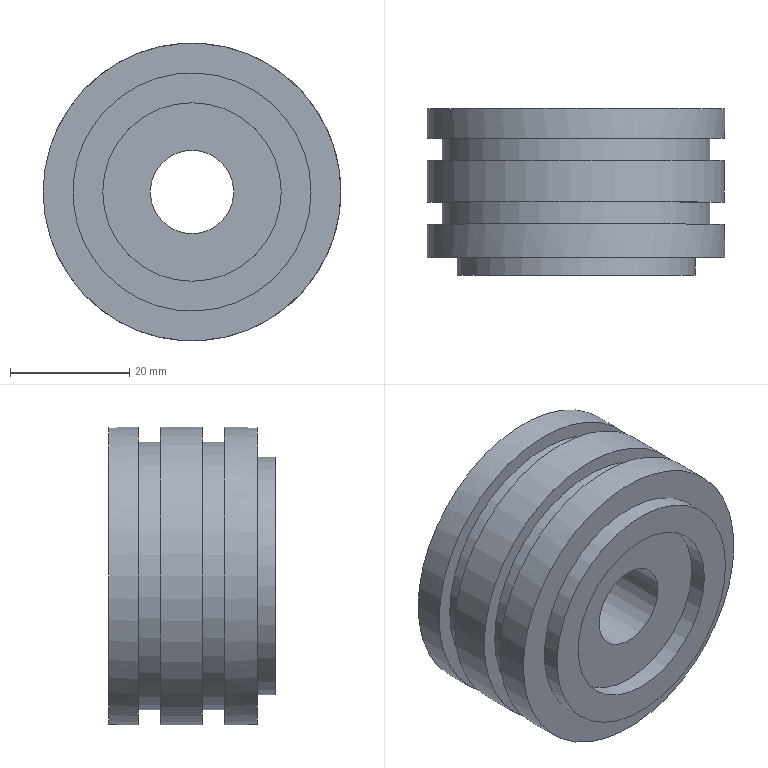Component | NX | PISTON | 1 solid | 18 faces | box 50 x 28 x 50 mm | volume 29970 mm3 | plane 9 | cylinder 8 | cone 1 | commonest cylinder face diameters 50 x3 45 x2 14 x1 40 x1 30 x1
STEP:
#1=CARTESIAN_POINT('',(0.,0.,0.));
#2=DIRECTION('',(0.,0.,1.));
#3=DIRECTION('',(1.,0.,0.));
#4=AXIS2_PLACEMENT_3D('',#1,#2,#3);
#5=CARTESIAN_POINT('',(-25.,44.,43.));
#6=VERTEX_POINT('',#5);
#7=CARTESIAN_POINT('',(25.,44.,43.));
#8=VERTEX_POINT('',#7);
#9=CARTESIAN_POINT('',(-0.,44.,43.));
#10=DIRECTION('',(0.,-1.,0.));
#11=DIRECTION('',(1.,0.,0.));
#12=AXIS2_PLACEMENT_3D('',#9,#10,#11);
#13=CIRCLE('',#12,25.);
#14=CARTESIAN_POINT('',(-0.,44.,43.));
#15=DIRECTION('',(0.,1.,0.));
#16=DIRECTION('',(-1.,0.,0.));
#17=AXIS2_PLACEMENT_3D('',#14,#15,#16);
#18=CYLINDRICAL_SURFACE('',#17,25.);
#19=CARTESIAN_POINT('',(9.425,0.));
#20=DIRECTION('',(-1.,0.));
#21=VECTOR('',#20,1.);
#22=LINE('',#19,#21);
#23=(GEOMETRIC_REPRESENTATION_CONTEXT(2)PARAMETRIC_REPRESENTATION_CONTEXT()REPRESENTATION_CONTEXT('',''));
#24=DEFINITIONAL_REPRESENTATION('',(#22),#23);
#25=PCURVE('',#18,#24);
#26=CARTESIAN_POINT('',(-0.,44.,43.));
#27=DIRECTION('',(0.,-1.,0.));
#28=DIRECTION('',(1.,0.,0.));
#29=AXIS2_PLACEMENT_3D('',#26,#27,#28);
#30=PLANE('',#29);
#31=CARTESIAN_POINT('',(0.,0.));
#32=DIRECTION('',(1.,0.));
#33=AXIS2_PLACEMENT_2D('',#31,#32);
#34=CIRCLE('',#33,25.);
#35=(GEOMETRIC_REPRESENTATION_CONTEXT(2)PARAMETRIC_REPRESENTATION_CONTEXT()REPRESENTATION_CONTEXT('',''));
#36=DEFINITIONAL_REPRESENTATION('',(#34),#35);
#37=PCURVE('',#30,#36);
#38=SURFACE_CURVE('',#13,(#25,#37),.PCURVE_S1.);
#39=EDGE_CURVE('',#6,#8,#38,.T.);
#40=ORIENTED_EDGE('',*,*,#39,.F.);
#41=CARTESIAN_POINT('',(-25.,49.6,43.));
#42=VERTEX_POINT('',#41);
#43=CARTESIAN_POINT('',(-25.,44.,43.));
#44=CARTESIAN_POINT('',(-25.,49.6,43.));
#45=B_SPLINE_CURVE_WITH_KNOTS('',1,(#43,#44),.UNSPECIFIED.,.F.,.F.,(2,2),(0.,5.6),.PIECEWISE_BEZIER_KNOTS.);
#46=CARTESIAN_POINT('',(6.283,0.));
#47=DIRECTION('',(0.,1.));
#48=VECTOR('',#47,1.);
#49=LINE('',#46,#48);
#50=(GEOMETRIC_REPRESENTATION_CONTEXT(2)PARAMETRIC_REPRESENTATION_CONTEXT()REPRESENTATION_CONTEXT('',''));
#51=DEFINITIONAL_REPRESENTATION('',(#49),#50);
#52=PCURVE('',#18,#51);
#53=CARTESIAN_POINT('',(0.,0.));
#54=DIRECTION('',(0.,1.));
#55=VECTOR('',#54,1.);
#56=LINE('',#53,#55);
#57=(GEOMETRIC_REPRESENTATION_CONTEXT(2)PARAMETRIC_REPRESENTATION_CONTEXT()REPRESENTATION_CONTEXT('',''));
#58=DEFINITIONAL_REPRESENTATION('',(#56),#57);
#59=PCURVE('',#18,#58);
#60=SEAM_CURVE('',#45,(#52,#59),.PCURVE_S1.);
#61=EDGE_CURVE('',#6,#42,#60,.T.);
#62=ORIENTED_EDGE('',*,*,#61,.T.);
#63=CARTESIAN_POINT('',(-0.,49.6,43.));
#64=DIRECTION('',(0.,1.,0.));
#65=DIRECTION('',(-1.,0.,0.));
#66=AXIS2_PLACEMENT_3D('',#63,#64,#65);
#67=CIRCLE('',#66,25.);
#68=CARTESIAN_POINT('',(0.,5.6));
#69=DIRECTION('',(1.,0.));
#70=VECTOR('',#69,1.);
#71=LINE('',#68,#70);
#72=(GEOMETRIC_REPRESENTATION_CONTEXT(2)PARAMETRIC_REPRESENTATION_CONTEXT()REPRESENTATION_CONTEXT('',''));
#73=DEFINITIONAL_REPRESENTATION('',(#71),#72);
#74=PCURVE('',#18,#73);
#75=CARTESIAN_POINT('',(-0.,49.6,43.));
#76=DIRECTION('',(0.,1.,0.));
#77=DIRECTION('',(-1.,0.,0.));
#78=AXIS2_PLACEMENT_3D('',#75,#76,#77);
#79=PLANE('',#78);
#80=CARTESIAN_POINT('',(0.,0.));
#81=DIRECTION('',(1.,0.));
#82=AXIS2_PLACEMENT_2D('',#80,#81);
#83=CIRCLE('',#82,25.);
#84=(GEOMETRIC_REPRESENTATION_CONTEXT(2)PARAMETRIC_REPRESENTATION_CONTEXT()REPRESENTATION_CONTEXT('',''));
#85=DEFINITIONAL_REPRESENTATION('',(#83),#84);
#86=PCURVE('',#79,#85);
#87=SURFACE_CURVE('',#67,(#74,#86),.PCURVE_S1.);
#88=EDGE_CURVE('',#42,#42,#87,.T.);
#89=ORIENTED_EDGE('',*,*,#88,.F.);
#90=ORIENTED_EDGE('',*,*,#61,.F.);
#91=CARTESIAN_POINT('',(-0.,44.,43.));
#92=DIRECTION('',(0.,-1.,0.));
#93=DIRECTION('',(1.,0.,0.));
#94=AXIS2_PLACEMENT_3D('',#91,#92,#93);
#95=CIRCLE('',#94,25.);
#96=CARTESIAN_POINT('',(3.142,0.));
#97=DIRECTION('',(-1.,0.));
#98=VECTOR('',#97,1.);
#99=LINE('',#96,#98);
#100=(GEOMETRIC_REPRESENTATION_CONTEXT(2)PARAMETRIC_REPRESENTATION_CONTEXT()REPRESENTATION_CONTEXT('',''));
#101=DEFINITIONAL_REPRESENTATION('',(#99),#100);
#102=PCURVE('',#18,#101);
#103=CARTESIAN_POINT('',(0.,0.));
#104=DIRECTION('',(1.,0.));
#105=AXIS2_PLACEMENT_2D('',#103,#104);
#106=CIRCLE('',#105,25.);
#107=(GEOMETRIC_REPRESENTATION_CONTEXT(2)PARAMETRIC_REPRESENTATION_CONTEXT()REPRESENTATION_CONTEXT('',''));
#108=DEFINITIONAL_REPRESENTATION('',(#106),#107);
#109=PCURVE('',#30,#108);
#110=SURFACE_CURVE('',#95,(#102,#109),.PCURVE_S1.);
#111=EDGE_CURVE('',#8,#6,#110,.T.);
#112=ORIENTED_EDGE('',*,*,#111,.F.);
#113=EDGE_LOOP('',(#40,#62,#89,#90,#112));
#114=FACE_BOUND('',#113,.T.);
#115=ADVANCED_FACE('',(#114),#18,.T.);
#116=CARTESIAN_POINT('',(-25.,53.3,43.));
#117=VERTEX_POINT('',#116);
#118=CARTESIAN_POINT('',(-0.,53.3,43.));
#119=DIRECTION('',(0.,1.,0.));
#120=DIRECTION('',(-1.,0.,0.));
#121=AXIS2_PLACEMENT_3D('',#118,#119,#120);
#122=CIRCLE('',#121,25.);
#123=CARTESIAN_POINT('',(-0.,44.,43.));
#124=DIRECTION('',(0.,1.,0.));
#125=DIRECTION('',(-1.,0.,0.));
#126=AXIS2_PLACEMENT_3D('',#123,#124,#125);
#127=CYLINDRICAL_SURFACE('',#126,25.);
#128=CARTESIAN_POINT('',(0.,9.3));
#129=DIRECTION('',(1.,0.));
#130=VECTOR('',#129,1.);
#131=LINE('',#128,#130);
#132=(GEOMETRIC_REPRESENTATION_CONTEXT(2)PARAMETRIC_REPRESENTATION_CONTEXT()REPRESENTATION_CONTEXT('',''));
#133=DEFINITIONAL_REPRESENTATION('',(#131),#132);
#134=PCURVE('',#127,#133);
#135=CARTESIAN_POINT('',(-0.,53.3,43.));
#136=DIRECTION('',(0.,1.,0.));
#137=DIRECTION('',(-1.,0.,0.));
#138=AXIS2_PLACEMENT_3D('',#135,#136,#137);
#139=PLANE('',#138);
#140=CARTESIAN_POINT('',(0.,0.));
#141=DIRECTION('',(1.,0.));
#142=AXIS2_PLACEMENT_2D('',#140,#141);
#143=CIRCLE('',#142,25.);
#144=(GEOMETRIC_REPRESENTATION_CONTEXT(2)PARAMETRIC_REPRESENTATION_CONTEXT()REPRESENTATION_CONTEXT('',''));
#145=DEFINITIONAL_REPRESENTATION('',(#143),#144);
#146=PCURVE('',#139,#145);
#147=SURFACE_CURVE('',#122,(#134,#146),.PCURVE_S1.);
#148=EDGE_CURVE('',#117,#117,#147,.T.);
#149=ORIENTED_EDGE('',*,*,#148,.T.);
#150=CARTESIAN_POINT('',(-25.,60.3,43.));
#151=VERTEX_POINT('',#150);
#152=CARTESIAN_POINT('',(-25.,53.3,43.));
#153=CARTESIAN_POINT('',(-25.,60.3,43.));
#154=B_SPLINE_CURVE_WITH_KNOTS('',1,(#152,#153),.UNSPECIFIED.,.F.,.F.,(2,2),(9.3,16.3),.PIECEWISE_BEZIER_KNOTS.);
#155=CARTESIAN_POINT('',(6.283,0.));
#156=DIRECTION('',(0.,1.));
#157=VECTOR('',#156,1.);
#158=LINE('',#155,#157);
#159=(GEOMETRIC_REPRESENTATION_CONTEXT(2)PARAMETRIC_REPRESENTATION_CONTEXT()REPRESENTATION_CONTEXT('',''));
#160=DEFINITIONAL_REPRESENTATION('',(#158),#159);
#161=PCURVE('',#127,#160);
#162=CARTESIAN_POINT('',(0.,0.));
#163=DIRECTION('',(0.,1.));
#164=VECTOR('',#163,1.);
#165=LINE('',#162,#164);
#166=(GEOMETRIC_REPRESENTATION_CONTEXT(2)PARAMETRIC_REPRESENTATION_CONTEXT()REPRESENTATION_CONTEXT('',''));
#167=DEFINITIONAL_REPRESENTATION('',(#165),#166);
#168=PCURVE('',#127,#167);
#169=SEAM_CURVE('',#154,(#161,#168),.PCURVE_S1.);
#170=EDGE_CURVE('',#117,#151,#169,.T.);
#171=ORIENTED_EDGE('',*,*,#170,.T.);
#172=CARTESIAN_POINT('',(-0.,60.3,43.));
#173=DIRECTION('',(0.,1.,0.));
#174=DIRECTION('',(-1.,0.,0.));
#175=AXIS2_PLACEMENT_3D('',#172,#173,#174);
#176=CIRCLE('',#175,25.);
#177=CARTESIAN_POINT('',(0.,16.3));
#178=DIRECTION('',(1.,0.));
#179=VECTOR('',#178,1.);
#180=LINE('',#177,#179);
#181=(GEOMETRIC_REPRESENTATION_CONTEXT(2)PARAMETRIC_REPRESENTATION_CONTEXT()REPRESENTATION_CONTEXT('',''));
#182=DEFINITIONAL_REPRESENTATION('',(#180),#181);
#183=PCURVE('',#127,#182);
#184=CARTESIAN_POINT('',(-0.,60.3,43.));
#185=DIRECTION('',(0.,1.,0.));
#186=DIRECTION('',(-1.,0.,0.));
#187=AXIS2_PLACEMENT_3D('',#184,#185,#186);
#188=PLANE('',#187);
#189=CARTESIAN_POINT('',(0.,0.));
#190=DIRECTION('',(1.,0.));
#191=AXIS2_PLACEMENT_2D('',#189,#190);
#192=CIRCLE('',#191,25.);
#193=(GEOMETRIC_REPRESENTATION_CONTEXT(2)PARAMETRIC_REPRESENTATION_CONTEXT()REPRESENTATION_CONTEXT('',''));
#194=DEFINITIONAL_REPRESENTATION('',(#192),#193);
#195=PCURVE('',#188,#194);
#196=SURFACE_CURVE('',#176,(#183,#195),.PCURVE_S1.);
#197=EDGE_CURVE('',#151,#151,#196,.T.);
#198=ORIENTED_EDGE('',*,*,#197,.F.);
#199=ORIENTED_EDGE('',*,*,#170,.F.);
#200=EDGE_LOOP('',(#149,#171,#198,#199));
#201=FACE_BOUND('',#200,.T.);
#202=ADVANCED_FACE('',(#201),#127,.T.);
#203=CARTESIAN_POINT('',(7.,44.,43.));
#204=VERTEX_POINT('',#203);
#205=CARTESIAN_POINT('',(-7.,44.,43.));
#206=VERTEX_POINT('',#205);
#207=CARTESIAN_POINT('',(-0.,44.,43.));
#208=DIRECTION('',(0.,1.,0.));
#209=DIRECTION('',(1.,0.,0.));
#210=AXIS2_PLACEMENT_3D('',#207,#208,#209);
#211=CIRCLE('',#210,7.);
#212=CARTESIAN_POINT('',(-0.,41.,43.));
#213=DIRECTION('',(0.,1.,0.));
#214=DIRECTION('',(-1.,0.,0.));
#215=AXIS2_PLACEMENT_3D('',#212,#213,#214);
#216=CYLINDRICAL_SURFACE('',#215,7.);
#217=CARTESIAN_POINT('',(3.142,3.));
#218=DIRECTION('',(1.,0.));
#219=VECTOR('',#218,1.);
#220=LINE('',#217,#219);
#221=(GEOMETRIC_REPRESENTATION_CONTEXT(2)PARAMETRIC_REPRESENTATION_CONTEXT()REPRESENTATION_CONTEXT('',''));
#222=DEFINITIONAL_REPRESENTATION('',(#220),#221);
#223=PCURVE('',#216,#222);
#224=CARTESIAN_POINT('',(-0.,44.,43.));
#225=DIRECTION('',(0.,-1.,0.));
#226=DIRECTION('',(1.,0.,0.));
#227=AXIS2_PLACEMENT_3D('',#224,#225,#226);
#228=PLANE('',#227);
#229=CARTESIAN_POINT('',(7.,0.));
#230=CARTESIAN_POINT('',(7.,-12.124));
#231=CARTESIAN_POINT('',(-3.5,-6.062));
#232=CARTESIAN_POINT('',(-14.,-0.));
#233=CARTESIAN_POINT('',(-3.5,6.062));
#234=CARTESIAN_POINT('',(7.,12.124));
#235=CARTESIAN_POINT('',(7.,0.));
#236=(BOUNDED_CURVE()B_SPLINE_CURVE(2,(#229,#230,#231,#232,#233,#234,#235),.UNSPECIFIED.,.T.,.F.)B_SPLINE_CURVE_WITH_KNOTS((1,2,2,2,2,1),(-2.094,0.,2.094,4.189,6.283,8.378),.UNSPECIFIED.)CURVE()GEOMETRIC_REPRESENTATION_ITEM()RATIONAL_B_SPLINE_CURVE((1.,0.5,1.,0.5,1.,0.5,1.))REPRESENTATION_ITEM(''));
#237=(GEOMETRIC_REPRESENTATION_CONTEXT(2)PARAMETRIC_REPRESENTATION_CONTEXT()REPRESENTATION_CONTEXT('',''));
#238=DEFINITIONAL_REPRESENTATION('',(#236),#237);
#239=PCURVE('',#228,#238);
#240=SURFACE_CURVE('',#211,(#223,#239),.PCURVE_S1.);
#241=EDGE_CURVE('',#204,#206,#240,.T.);
#242=ORIENTED_EDGE('',*,*,#241,.T.);
#243=CARTESIAN_POINT('',(-7.,54.,43.));
#244=VERTEX_POINT('',#243);
#245=CARTESIAN_POINT('',(-7.,44.,43.));
#246=CARTESIAN_POINT('',(-7.,54.,43.));
#247=B_SPLINE_CURVE_WITH_KNOTS('',1,(#245,#246),.UNSPECIFIED.,.F.,.F.,(2,2),(3.,13.),.PIECEWISE_BEZIER_KNOTS.);
#248=CARTESIAN_POINT('',(6.283,0.));
#249=DIRECTION('',(0.,1.));
#250=VECTOR('',#249,1.);
#251=LINE('',#248,#250);
#252=(GEOMETRIC_REPRESENTATION_CONTEXT(2)PARAMETRIC_REPRESENTATION_CONTEXT()REPRESENTATION_CONTEXT('',''));
#253=DEFINITIONAL_REPRESENTATION('',(#251),#252);
#254=PCURVE('',#216,#253);
#255=CARTESIAN_POINT('',(0.,0.));
#256=DIRECTION('',(0.,1.));
#257=VECTOR('',#256,1.);
#258=LINE('',#255,#257);
#259=(GEOMETRIC_REPRESENTATION_CONTEXT(2)PARAMETRIC_REPRESENTATION_CONTEXT()REPRESENTATION_CONTEXT('',''));
#260=DEFINITIONAL_REPRESENTATION('',(#258),#259);
#261=PCURVE('',#216,#260);
#262=SEAM_CURVE('',#247,(#254,#261),.PCURVE_S1.);
#263=EDGE_CURVE('',#206,#244,#262,.T.);
#264=ORIENTED_EDGE('',*,*,#263,.T.);
#265=CARTESIAN_POINT('',(-0.,54.,43.));
#266=DIRECTION('',(0.,-1.,0.));
#267=DIRECTION('',(-1.,0.,0.));
#268=AXIS2_PLACEMENT_3D('',#265,#266,#267);
#269=CIRCLE('',#268,7.);
#270=CARTESIAN_POINT('',(6.283,13.));
#271=DIRECTION('',(-1.,0.));
#272=VECTOR('',#271,1.);
#273=LINE('',#270,#272);
#274=(GEOMETRIC_REPRESENTATION_CONTEXT(2)PARAMETRIC_REPRESENTATION_CONTEXT()REPRESENTATION_CONTEXT('',''));
#275=DEFINITIONAL_REPRESENTATION('',(#273),#274);
#276=PCURVE('',#216,#275);
#277=CARTESIAN_POINT('',(-0.,54.,43.));
#278=DIRECTION('',(0.,1.,0.));
#279=DIRECTION('',(-1.,0.,0.));
#280=AXIS2_PLACEMENT_3D('',#277,#278,#279);
#281=PLANE('',#280);
#282=CARTESIAN_POINT('',(7.,0.));
#283=CARTESIAN_POINT('',(7.,-12.124));
#284=CARTESIAN_POINT('',(-3.5,-6.062));
#285=CARTESIAN_POINT('',(-14.,-0.));
#286=CARTESIAN_POINT('',(-3.5,6.062));
#287=CARTESIAN_POINT('',(7.,12.124));
#288=CARTESIAN_POINT('',(7.,0.));
#289=(BOUNDED_CURVE()B_SPLINE_CURVE(2,(#282,#283,#284,#285,#286,#287,#288),.UNSPECIFIED.,.T.,.F.)B_SPLINE_CURVE_WITH_KNOTS((1,2,2,2,2,1),(-2.094,0.,2.094,4.189,6.283,8.378),.UNSPECIFIED.)CURVE()GEOMETRIC_REPRESENTATION_ITEM()RATIONAL_B_SPLINE_CURVE((1.,0.5,1.,0.5,1.,0.5,1.))REPRESENTATION_ITEM(''));
#290=(GEOMETRIC_REPRESENTATION_CONTEXT(2)PARAMETRIC_REPRESENTATION_CONTEXT()REPRESENTATION_CONTEXT('',''));
#291=DEFINITIONAL_REPRESENTATION('',(#289),#290);
#292=PCURVE('',#281,#291);
#293=SURFACE_CURVE('',#269,(#276,#292),.PCURVE_S1.);
#294=EDGE_CURVE('',#244,#244,#293,.T.);
#295=ORIENTED_EDGE('',*,*,#294,.T.);
#296=ORIENTED_EDGE('',*,*,#263,.F.);
#297=CARTESIAN_POINT('',(-0.,44.,43.));
#298=DIRECTION('',(0.,1.,0.));
#299=DIRECTION('',(1.,0.,0.));
#300=AXIS2_PLACEMENT_3D('',#297,#298,#299);
#301=CIRCLE('',#300,7.);
#302=CARTESIAN_POINT('',(-3.142,3.));
#303=DIRECTION('',(1.,0.));
#304=VECTOR('',#303,1.);
#305=LINE('',#302,#304);
#306=(GEOMETRIC_REPRESENTATION_CONTEXT(2)PARAMETRIC_REPRESENTATION_CONTEXT()REPRESENTATION_CONTEXT('',''));
#307=DEFINITIONAL_REPRESENTATION('',(#305),#306);
#308=PCURVE('',#216,#307);
#309=CARTESIAN_POINT('',(7.,0.));
#310=CARTESIAN_POINT('',(7.,-12.124));
#311=CARTESIAN_POINT('',(-3.5,-6.062));
#312=CARTESIAN_POINT('',(-14.,-0.));
#313=CARTESIAN_POINT('',(-3.5,6.062));
#314=CARTESIAN_POINT('',(7.,12.124));
#315=CARTESIAN_POINT('',(7.,0.));
#316=(BOUNDED_CURVE()B_SPLINE_CURVE(2,(#309,#310,#311,#312,#313,#314,#315),.UNSPECIFIED.,.T.,.F.)B_SPLINE_CURVE_WITH_KNOTS((1,2,2,2,2,1),(-2.094,0.,2.094,4.189,6.283,8.378),.UNSPECIFIED.)CURVE()GEOMETRIC_REPRESENTATION_ITEM()RATIONAL_B_SPLINE_CURVE((1.,0.5,1.,0.5,1.,0.5,1.))REPRESENTATION_ITEM(''));
#317=(GEOMETRIC_REPRESENTATION_CONTEXT(2)PARAMETRIC_REPRESENTATION_CONTEXT()REPRESENTATION_CONTEXT('',''));
#318=DEFINITIONAL_REPRESENTATION('',(#316),#317);
#319=PCURVE('',#228,#318);
#320=SURFACE_CURVE('',#301,(#308,#319),.PCURVE_S1.);
#321=EDGE_CURVE('',#206,#204,#320,.T.);
#322=ORIENTED_EDGE('',*,*,#321,.T.);
#323=EDGE_LOOP('',(#242,#264,#295,#296,#322));
#324=FACE_BOUND('',#323,.F.);
#325=ADVANCED_FACE('',(#324),#216,.F.);
#326=CARTESIAN_POINT('',(-25.,64.,43.));
#327=VERTEX_POINT('',#326);
#328=CARTESIAN_POINT('',(-0.,64.,43.));
#329=DIRECTION('',(0.,1.,0.));
#330=DIRECTION('',(-1.,0.,0.));
#331=AXIS2_PLACEMENT_3D('',#328,#329,#330);
#332=CIRCLE('',#331,25.);
#333=CARTESIAN_POINT('',(-0.,44.,43.));
#334=DIRECTION('',(0.,1.,0.));
#335=DIRECTION('',(-1.,0.,0.));
#336=AXIS2_PLACEMENT_3D('',#333,#334,#335);
#337=CYLINDRICAL_SURFACE('',#336,25.);
#338=CARTESIAN_POINT('',(0.,20.));
#339=DIRECTION('',(1.,0.));
#340=VECTOR('',#339,1.);
#341=LINE('',#338,#340);
#342=(GEOMETRIC_REPRESENTATION_CONTEXT(2)PARAMETRIC_REPRESENTATION_CONTEXT()REPRESENTATION_CONTEXT('',''));
#343=DEFINITIONAL_REPRESENTATION('',(#341),#342);
#344=PCURVE('',#337,#343);
#345=CARTESIAN_POINT('',(-0.,64.,43.));
#346=DIRECTION('',(0.,1.,0.));
#347=DIRECTION('',(-1.,0.,0.));
#348=AXIS2_PLACEMENT_3D('',#345,#346,#347);
#349=PLANE('',#348);
#350=CARTESIAN_POINT('',(0.,0.));
#351=DIRECTION('',(1.,0.));
#352=AXIS2_PLACEMENT_2D('',#350,#351);
#353=CIRCLE('',#352,25.);
#354=(GEOMETRIC_REPRESENTATION_CONTEXT(2)PARAMETRIC_REPRESENTATION_CONTEXT()REPRESENTATION_CONTEXT('',''));
#355=DEFINITIONAL_REPRESENTATION('',(#353),#354);
#356=PCURVE('',#349,#355);
#357=SURFACE_CURVE('',#332,(#344,#356),.PCURVE_S1.);
#358=EDGE_CURVE('',#327,#327,#357,.T.);
#359=ORIENTED_EDGE('',*,*,#358,.T.);
#360=CARTESIAN_POINT('',(-25.,69.,43.));
#361=VERTEX_POINT('',#360);
#362=CARTESIAN_POINT('',(-25.,64.,43.));
#363=CARTESIAN_POINT('',(-25.,69.,43.));
#364=B_SPLINE_CURVE_WITH_KNOTS('',1,(#362,#363),.UNSPECIFIED.,.F.,.F.,(2,2),(20.,25.),.PIECEWISE_BEZIER_KNOTS.);
#365=CARTESIAN_POINT('',(6.283,0.));
#366=DIRECTION('',(0.,1.));
#367=VECTOR('',#366,1.);
#368=LINE('',#365,#367);
#369=(GEOMETRIC_REPRESENTATION_CONTEXT(2)PARAMETRIC_REPRESENTATION_CONTEXT()REPRESENTATION_CONTEXT('',''));
#370=DEFINITIONAL_REPRESENTATION('',(#368),#369);
#371=PCURVE('',#337,#370);
#372=CARTESIAN_POINT('',(0.,0.));
#373=DIRECTION('',(0.,1.));
#374=VECTOR('',#373,1.);
#375=LINE('',#372,#374);
#376=(GEOMETRIC_REPRESENTATION_CONTEXT(2)PARAMETRIC_REPRESENTATION_CONTEXT()REPRESENTATION_CONTEXT('',''));
#377=DEFINITIONAL_REPRESENTATION('',(#375),#376);
#378=PCURVE('',#337,#377);
#379=SEAM_CURVE('',#364,(#371,#378),.PCURVE_S1.);
#380=EDGE_CURVE('',#327,#361,#379,.T.);
#381=ORIENTED_EDGE('',*,*,#380,.T.);
#382=CARTESIAN_POINT('',(25.,69.,43.));
#383=VERTEX_POINT('',#382);
#384=CARTESIAN_POINT('',(-0.,69.,43.));
#385=DIRECTION('',(0.,-1.,0.));
#386=DIRECTION('',(1.,0.,0.));
#387=AXIS2_PLACEMENT_3D('',#384,#385,#386);
#388=CIRCLE('',#387,25.);
#389=CARTESIAN_POINT('',(9.425,25.));
#390=DIRECTION('',(-1.,0.));
#391=VECTOR('',#390,1.);
#392=LINE('',#389,#391);
#393=(GEOMETRIC_REPRESENTATION_CONTEXT(2)PARAMETRIC_REPRESENTATION_CONTEXT()REPRESENTATION_CONTEXT('',''));
#394=DEFINITIONAL_REPRESENTATION('',(#392),#393);
#395=PCURVE('',#337,#394);
#396=CARTESIAN_POINT('',(-0.,69.,43.));
#397=DIRECTION('',(0.,-1.,0.));
#398=DIRECTION('',(1.,0.,0.));
#399=AXIS2_PLACEMENT_3D('',#396,#397,#398);
#400=PLANE('',#399);
#401=CARTESIAN_POINT('',(0.,0.));
#402=DIRECTION('',(1.,0.));
#403=AXIS2_PLACEMENT_2D('',#401,#402);
#404=CIRCLE('',#403,25.);
#405=(GEOMETRIC_REPRESENTATION_CONTEXT(2)PARAMETRIC_REPRESENTATION_CONTEXT()REPRESENTATION_CONTEXT('',''));
#406=DEFINITIONAL_REPRESENTATION('',(#404),#405);
#407=PCURVE('',#400,#406);
#408=SURFACE_CURVE('',#388,(#395,#407),.PCURVE_S1.);
#409=EDGE_CURVE('',#361,#383,#408,.T.);
#410=ORIENTED_EDGE('',*,*,#409,.T.);
#411=CARTESIAN_POINT('',(-0.,69.,43.));
#412=DIRECTION('',(0.,-1.,0.));
#413=DIRECTION('',(1.,0.,0.));
#414=AXIS2_PLACEMENT_3D('',#411,#412,#413);
#415=CIRCLE('',#414,25.);
#416=CARTESIAN_POINT('',(3.142,25.));
#417=DIRECTION('',(-1.,0.));
#418=VECTOR('',#417,1.);
#419=LINE('',#416,#418);
#420=(GEOMETRIC_REPRESENTATION_CONTEXT(2)PARAMETRIC_REPRESENTATION_CONTEXT()REPRESENTATION_CONTEXT('',''));
#421=DEFINITIONAL_REPRESENTATION('',(#419),#420);
#422=PCURVE('',#337,#421);
#423=CARTESIAN_POINT('',(0.,0.));
#424=DIRECTION('',(1.,0.));
#425=AXIS2_PLACEMENT_2D('',#423,#424);
#426=CIRCLE('',#425,25.);
#427=(GEOMETRIC_REPRESENTATION_CONTEXT(2)PARAMETRIC_REPRESENTATION_CONTEXT()REPRESENTATION_CONTEXT('',''));
#428=DEFINITIONAL_REPRESENTATION('',(#426),#427);
#429=PCURVE('',#400,#428);
#430=SURFACE_CURVE('',#415,(#422,#429),.PCURVE_S1.);
#431=EDGE_CURVE('',#383,#361,#430,.T.);
#432=ORIENTED_EDGE('',*,*,#431,.T.);
#433=ORIENTED_EDGE('',*,*,#380,.F.);
#434=EDGE_LOOP('',(#359,#381,#410,#432,#433));
#435=FACE_BOUND('',#434,.T.);
#436=ADVANCED_FACE('',(#435),#337,.T.);
#437=CARTESIAN_POINT('',(20.,44.,43.));
#438=VERTEX_POINT('',#437);
#439=CARTESIAN_POINT('',(-0.,44.,43.));
#440=DIRECTION('',(0.,-1.,0.));
#441=DIRECTION('',(1.,0.,0.));
#442=AXIS2_PLACEMENT_3D('',#439,#440,#441);
#443=CIRCLE('',#442,20.);
#444=CARTESIAN_POINT('',(0.,0.));
#445=DIRECTION('',(1.,0.));
#446=AXIS2_PLACEMENT_2D('',#444,#445);
#447=CIRCLE('',#446,20.);
#448=(GEOMETRIC_REPRESENTATION_CONTEXT(2)PARAMETRIC_REPRESENTATION_CONTEXT()REPRESENTATION_CONTEXT('',''));
#449=DEFINITIONAL_REPRESENTATION('',(#447),#448);
#450=PCURVE('',#30,#449);
#451=CARTESIAN_POINT('',(-0.,41.,43.));
#452=DIRECTION('',(0.,1.,0.));
#453=DIRECTION('',(-1.,0.,0.));
#454=AXIS2_PLACEMENT_3D('',#451,#452,#453);
#455=CYLINDRICAL_SURFACE('',#454,20.);
#456=CARTESIAN_POINT('',(9.425,3.));
#457=DIRECTION('',(-1.,0.));
#458=VECTOR('',#457,1.);
#459=LINE('',#456,#458);
#460=(GEOMETRIC_REPRESENTATION_CONTEXT(2)PARAMETRIC_REPRESENTATION_CONTEXT()REPRESENTATION_CONTEXT('',''));
#461=DEFINITIONAL_REPRESENTATION('',(#459),#460);
#462=PCURVE('',#455,#461);
#463=SURFACE_CURVE('',#443,(#450,#462),.PCURVE_S1.);
#464=EDGE_CURVE('',#438,#438,#463,.T.);
#465=ORIENTED_EDGE('',*,*,#464,.F.);
#466=EDGE_LOOP('',(#465));
#467=FACE_BOUND('',#466,.T.);
#468=ORIENTED_EDGE('',*,*,#111,.T.);
#469=ORIENTED_EDGE('',*,*,#39,.T.);
#470=EDGE_LOOP('',(#468,#469));
#471=FACE_BOUND('',#470,.T.);
#472=ADVANCED_FACE('',(#467,#471),#30,.T.);
#473=CARTESIAN_POINT('',(20.,69.,43.));
#474=VERTEX_POINT('',#473);
#475=CARTESIAN_POINT('',(-20.,69.,43.));
#476=VERTEX_POINT('',#475);
#477=CARTESIAN_POINT('',(-0.,69.,43.));
#478=DIRECTION('',(0.,1.,0.));
#479=DIRECTION('',(1.,0.,0.));
#480=AXIS2_PLACEMENT_3D('',#477,#478,#479);
#481=CIRCLE('',#480,20.);
#482=CARTESIAN_POINT('',(20.,0.));
#483=CARTESIAN_POINT('',(20.,-34.641));
#484=CARTESIAN_POINT('',(-10.,-17.321));
#485=CARTESIAN_POINT('',(-40.,-0.));
#486=CARTESIAN_POINT('',(-10.,17.321));
#487=CARTESIAN_POINT('',(20.,34.641));
#488=CARTESIAN_POINT('',(20.,0.));
#489=(BOUNDED_CURVE()B_SPLINE_CURVE(2,(#482,#483,#484,#485,#486,#487,#488),.UNSPECIFIED.,.T.,.F.)B_SPLINE_CURVE_WITH_KNOTS((1,2,2,2,2,1),(-2.094,0.,2.094,4.189,6.283,8.378),.UNSPECIFIED.)CURVE()GEOMETRIC_REPRESENTATION_ITEM()RATIONAL_B_SPLINE_CURVE((1.,0.5,1.,0.5,1.,0.5,1.))REPRESENTATION_ITEM(''));
#490=(GEOMETRIC_REPRESENTATION_CONTEXT(2)PARAMETRIC_REPRESENTATION_CONTEXT()REPRESENTATION_CONTEXT('',''));
#491=DEFINITIONAL_REPRESENTATION('',(#489),#490);
#492=PCURVE('',#400,#491);
#493=CARTESIAN_POINT('',(-0.,69.,43.));
#494=DIRECTION('',(0.,1.,0.));
#495=DIRECTION('',(-1.,0.,0.));
#496=AXIS2_PLACEMENT_3D('',#493,#494,#495);
#497=CONICAL_SURFACE('',#496,20.,0.1745);
#498=CARTESIAN_POINT('',(3.142,0.));
#499=DIRECTION('',(1.,0.));
#500=VECTOR('',#499,1.);
#501=LINE('',#498,#500);
#502=(GEOMETRIC_REPRESENTATION_CONTEXT(2)PARAMETRIC_REPRESENTATION_CONTEXT()REPRESENTATION_CONTEXT('',''));
#503=DEFINITIONAL_REPRESENTATION('',(#501),#502);
#504=PCURVE('',#497,#503);
#505=SURFACE_CURVE('',#481,(#492,#504),.PCURVE_S1.);
#506=EDGE_CURVE('',#474,#476,#505,.T.);
#507=ORIENTED_EDGE('',*,*,#506,.F.);
#508=CARTESIAN_POINT('',(-0.,69.,43.));
#509=DIRECTION('',(0.,1.,0.));
#510=DIRECTION('',(1.,0.,0.));
#511=AXIS2_PLACEMENT_3D('',#508,#509,#510);
#512=CIRCLE('',#511,20.);
#513=CARTESIAN_POINT('',(20.,0.));
#514=CARTESIAN_POINT('',(20.,-34.641));
#515=CARTESIAN_POINT('',(-10.,-17.321));
#516=CARTESIAN_POINT('',(-40.,-0.));
#517=CARTESIAN_POINT('',(-10.,17.321));
#518=CARTESIAN_POINT('',(20.,34.641));
#519=CARTESIAN_POINT('',(20.,0.));
#520=(BOUNDED_CURVE()B_SPLINE_CURVE(2,(#513,#514,#515,#516,#517,#518,#519),.UNSPECIFIED.,.T.,.F.)B_SPLINE_CURVE_WITH_KNOTS((1,2,2,2,2,1),(-2.094,0.,2.094,4.189,6.283,8.378),.UNSPECIFIED.)CURVE()GEOMETRIC_REPRESENTATION_ITEM()RATIONAL_B_SPLINE_CURVE((1.,0.5,1.,0.5,1.,0.5,1.))REPRESENTATION_ITEM(''));
#521=(GEOMETRIC_REPRESENTATION_CONTEXT(2)PARAMETRIC_REPRESENTATION_CONTEXT()REPRESENTATION_CONTEXT('',''));
#522=DEFINITIONAL_REPRESENTATION('',(#520),#521);
#523=PCURVE('',#400,#522);
#524=CARTESIAN_POINT('',(-3.142,0.));
#525=DIRECTION('',(1.,0.));
#526=VECTOR('',#525,1.);
#527=LINE('',#524,#526);
#528=(GEOMETRIC_REPRESENTATION_CONTEXT(2)PARAMETRIC_REPRESENTATION_CONTEXT()REPRESENTATION_CONTEXT('',''));
#529=DEFINITIONAL_REPRESENTATION('',(#527),#528);
#530=PCURVE('',#497,#529);
#531=SURFACE_CURVE('',#512,(#523,#530),.PCURVE_S1.);
#532=EDGE_CURVE('',#476,#474,#531,.T.);
#533=ORIENTED_EDGE('',*,*,#532,.F.);
#534=EDGE_LOOP('',(#507,#533));
#535=FACE_BOUND('',#534,.T.);
#536=ORIENTED_EDGE('',*,*,#431,.F.);
#537=ORIENTED_EDGE('',*,*,#409,.F.);
#538=EDGE_LOOP('',(#536,#537));
#539=FACE_BOUND('',#538,.T.);
#540=ADVANCED_FACE('',(#535,#539),#400,.F.);
#541=CARTESIAN_POINT('',(20.,41.,43.));
#542=VERTEX_POINT('',#541);
#543=CARTESIAN_POINT('',(-0.,41.,43.));
#544=DIRECTION('',(0.,-1.,0.));
#545=DIRECTION('',(1.,0.,0.));
#546=AXIS2_PLACEMENT_3D('',#543,#544,#545);
#547=CIRCLE('',#546,20.);
#548=CARTESIAN_POINT('',(9.425,0.));
#549=DIRECTION('',(-1.,0.));
#550=VECTOR('',#549,1.);
#551=LINE('',#548,#550);
#552=(GEOMETRIC_REPRESENTATION_CONTEXT(2)PARAMETRIC_REPRESENTATION_CONTEXT()REPRESENTATION_CONTEXT('',''));
#553=DEFINITIONAL_REPRESENTATION('',(#551),#552);
#554=PCURVE('',#455,#553);
#555=CARTESIAN_POINT('',(-0.,41.,43.));
#556=DIRECTION('',(0.,-1.,0.));
#557=DIRECTION('',(1.,0.,0.));
#558=AXIS2_PLACEMENT_3D('',#555,#556,#557);
#559=PLANE('',#558);
#560=CARTESIAN_POINT('',(0.,0.));
#561=DIRECTION('',(1.,0.));
#562=AXIS2_PLACEMENT_2D('',#560,#561);
#563=CIRCLE('',#562,20.);
#564=(GEOMETRIC_REPRESENTATION_CONTEXT(2)PARAMETRIC_REPRESENTATION_CONTEXT()REPRESENTATION_CONTEXT('',''));
#565=DEFINITIONAL_REPRESENTATION('',(#563),#564);
#566=PCURVE('',#559,#565);
#567=SURFACE_CURVE('',#547,(#554,#566),.PCURVE_S1.);
#568=EDGE_CURVE('',#542,#542,#567,.T.);
#569=ORIENTED_EDGE('',*,*,#568,.F.);
#570=CARTESIAN_POINT('',(20.,41.,43.));
#571=CARTESIAN_POINT('',(20.,44.,43.));
#572=B_SPLINE_CURVE_WITH_KNOTS('',1,(#570,#571),.UNSPECIFIED.,.F.,.F.,(2,2),(0.,3.),.PIECEWISE_BEZIER_KNOTS.);
#573=CARTESIAN_POINT('',(9.425,0.));
#574=DIRECTION('',(0.,1.));
#575=VECTOR('',#574,1.);
#576=LINE('',#573,#575);
#577=(GEOMETRIC_REPRESENTATION_CONTEXT(2)PARAMETRIC_REPRESENTATION_CONTEXT()REPRESENTATION_CONTEXT('',''));
#578=DEFINITIONAL_REPRESENTATION('',(#576),#577);
#579=PCURVE('',#455,#578);
#580=CARTESIAN_POINT('',(3.142,0.));
#581=DIRECTION('',(0.,1.));
#582=VECTOR('',#581,1.);
#583=LINE('',#580,#582);
#584=(GEOMETRIC_REPRESENTATION_CONTEXT(2)PARAMETRIC_REPRESENTATION_CONTEXT()REPRESENTATION_CONTEXT('',''));
#585=DEFINITIONAL_REPRESENTATION('',(#583),#584);
#586=PCURVE('',#455,#585);
#587=SEAM_CURVE('',#572,(#579,#586),.PCURVE_S1.);
#588=EDGE_CURVE('',#542,#438,#587,.T.);
#589=ORIENTED_EDGE('',*,*,#588,.T.);
#590=ORIENTED_EDGE('',*,*,#464,.T.);
#591=ORIENTED_EDGE('',*,*,#588,.F.);
#592=EDGE_LOOP('',(#569,#589,#590,#591));
#593=FACE_BOUND('',#592,.T.);
#594=ADVANCED_FACE('',(#593),#455,.T.);
#595=CARTESIAN_POINT('',(15.,41.,43.));
#596=VERTEX_POINT('',#595);
#597=CARTESIAN_POINT('',(-0.,41.,43.));
#598=DIRECTION('',(0.,-1.,0.));
#599=DIRECTION('',(1.,0.,0.));
#600=AXIS2_PLACEMENT_3D('',#597,#598,#599);
#601=CIRCLE('',#600,15.);
#602=CARTESIAN_POINT('',(0.,0.));
#603=DIRECTION('',(1.,0.));
#604=AXIS2_PLACEMENT_2D('',#602,#603);
#605=CIRCLE('',#604,15.);
#606=(GEOMETRIC_REPRESENTATION_CONTEXT(2)PARAMETRIC_REPRESENTATION_CONTEXT()REPRESENTATION_CONTEXT('',''));
#607=DEFINITIONAL_REPRESENTATION('',(#605),#606);
#608=PCURVE('',#559,#607);
#609=CARTESIAN_POINT('',(-0.,44.,43.));
#610=DIRECTION('',(0.,-1.,0.));
#611=DIRECTION('',(1.,0.,0.));
#612=AXIS2_PLACEMENT_3D('',#609,#610,#611);
#613=CYLINDRICAL_SURFACE('',#612,15.);
#614=CARTESIAN_POINT('',(0.,3.));
#615=DIRECTION('',(1.,0.));
#616=VECTOR('',#615,1.);
#617=LINE('',#614,#616);
#618=(GEOMETRIC_REPRESENTATION_CONTEXT(2)PARAMETRIC_REPRESENTATION_CONTEXT()REPRESENTATION_CONTEXT('',''));
#619=DEFINITIONAL_REPRESENTATION('',(#617),#618);
#620=PCURVE('',#613,#619);
#621=SURFACE_CURVE('',#601,(#608,#620),.PCURVE_S1.);
#622=EDGE_CURVE('',#596,#596,#621,.T.);
#623=ORIENTED_EDGE('',*,*,#622,.F.);
#624=EDGE_LOOP('',(#623));
#625=FACE_BOUND('',#624,.T.);
#626=ORIENTED_EDGE('',*,*,#568,.T.);
#627=EDGE_LOOP('',(#626));
#628=FACE_BOUND('',#627,.T.);
#629=ADVANCED_FACE('',(#625,#628),#559,.T.);
#630=CARTESIAN_POINT('',(15.,44.,43.));
#631=VERTEX_POINT('',#630);
#632=CARTESIAN_POINT('',(-0.,44.,43.));
#633=DIRECTION('',(0.,1.,0.));
#634=DIRECTION('',(1.,0.,0.));
#635=AXIS2_PLACEMENT_3D('',#632,#633,#634);
#636=CIRCLE('',#635,15.);
#637=CARTESIAN_POINT('',(15.,0.));
#638=CARTESIAN_POINT('',(15.,-25.981));
#639=CARTESIAN_POINT('',(-7.5,-12.99));
#640=CARTESIAN_POINT('',(-30.,-0.));
#641=CARTESIAN_POINT('',(-7.5,12.99));
#642=CARTESIAN_POINT('',(15.,25.981));
#643=CARTESIAN_POINT('',(15.,0.));
#644=(BOUNDED_CURVE()B_SPLINE_CURVE(2,(#637,#638,#639,#640,#641,#642,#643),.UNSPECIFIED.,.T.,.F.)B_SPLINE_CURVE_WITH_KNOTS((1,2,2,2,2,1),(-2.094,0.,2.094,4.189,6.283,8.378),.UNSPECIFIED.)CURVE()GEOMETRIC_REPRESENTATION_ITEM()RATIONAL_B_SPLINE_CURVE((1.,0.5,1.,0.5,1.,0.5,1.))REPRESENTATION_ITEM(''));
#645=(GEOMETRIC_REPRESENTATION_CONTEXT(2)PARAMETRIC_REPRESENTATION_CONTEXT()REPRESENTATION_CONTEXT('',''));
#646=DEFINITIONAL_REPRESENTATION('',(#644),#645);
#647=PCURVE('',#228,#646);
#648=CARTESIAN_POINT('',(6.283,0.));
#649=DIRECTION('',(-1.,0.));
#650=VECTOR('',#649,1.);
#651=LINE('',#648,#650);
#652=(GEOMETRIC_REPRESENTATION_CONTEXT(2)PARAMETRIC_REPRESENTATION_CONTEXT()REPRESENTATION_CONTEXT('',''));
#653=DEFINITIONAL_REPRESENTATION('',(#651),#652);
#654=PCURVE('',#613,#653);
#655=SURFACE_CURVE('',#636,(#647,#654),.PCURVE_S1.);
#656=EDGE_CURVE('',#631,#631,#655,.T.);
#657=ORIENTED_EDGE('',*,*,#656,.F.);
#658=EDGE_LOOP('',(#657));
#659=FACE_BOUND('',#658,.T.);
#660=ORIENTED_EDGE('',*,*,#241,.T.);
#661=ORIENTED_EDGE('',*,*,#321,.T.);
#662=EDGE_LOOP('',(#660,#661));
#663=FACE_BOUND('',#662,.T.);
#664=ADVANCED_FACE('',(#659,#663),#228,.T.);
#665=ORIENTED_EDGE('',*,*,#656,.F.);
#666=CARTESIAN_POINT('',(15.,44.,43.));
#667=CARTESIAN_POINT('',(15.,41.,43.));
#668=B_SPLINE_CURVE_WITH_KNOTS('',1,(#666,#667),.UNSPECIFIED.,.F.,.F.,(2,2),(0.,3.),.PIECEWISE_BEZIER_KNOTS.);
#669=CARTESIAN_POINT('',(6.283,0.));
#670=DIRECTION('',(0.,1.));
#671=VECTOR('',#670,1.);
#672=LINE('',#669,#671);
#673=(GEOMETRIC_REPRESENTATION_CONTEXT(2)PARAMETRIC_REPRESENTATION_CONTEXT()REPRESENTATION_CONTEXT('',''));
#674=DEFINITIONAL_REPRESENTATION('',(#672),#673);
#675=PCURVE('',#613,#674);
#676=CARTESIAN_POINT('',(0.,0.));
#677=DIRECTION('',(0.,1.));
#678=VECTOR('',#677,1.);
#679=LINE('',#676,#678);
#680=(GEOMETRIC_REPRESENTATION_CONTEXT(2)PARAMETRIC_REPRESENTATION_CONTEXT()REPRESENTATION_CONTEXT('',''));
#681=DEFINITIONAL_REPRESENTATION('',(#679),#680);
#682=PCURVE('',#613,#681);
#683=SEAM_CURVE('',#668,(#675,#682),.PCURVE_S1.);
#684=EDGE_CURVE('',#631,#596,#683,.T.);
#685=ORIENTED_EDGE('',*,*,#684,.T.);
#686=ORIENTED_EDGE('',*,*,#622,.F.);
#687=ORIENTED_EDGE('',*,*,#684,.F.);
#688=EDGE_LOOP('',(#665,#685,#686,#687));
#689=FACE_BOUND('',#688,.F.);
#690=ADVANCED_FACE('',(#689),#613,.F.);
#691=CARTESIAN_POINT('',(-17.355,54.,43.));
#692=VERTEX_POINT('',#691);
#693=CARTESIAN_POINT('',(-0.,54.,43.));
#694=DIRECTION('',(0.,-1.,0.));
#695=DIRECTION('',(-1.,0.,0.));
#696=AXIS2_PLACEMENT_3D('',#693,#694,#695);
#697=CIRCLE('',#696,17.355);
#698=CARTESIAN_POINT('',(17.355,0.));
#699=CARTESIAN_POINT('',(17.355,-30.06));
#700=CARTESIAN_POINT('',(-8.678,-15.03));
#701=CARTESIAN_POINT('',(-34.71,-0.));
#702=CARTESIAN_POINT('',(-8.678,15.03));
#703=CARTESIAN_POINT('',(17.355,30.06));
#704=CARTESIAN_POINT('',(17.355,0.));
#705=(BOUNDED_CURVE()B_SPLINE_CURVE(2,(#698,#699,#700,#701,#702,#703,#704),.UNSPECIFIED.,.T.,.F.)B_SPLINE_CURVE_WITH_KNOTS((1,2,2,2,2,1),(-2.094,0.,2.094,4.189,6.283,8.378),.UNSPECIFIED.)CURVE()GEOMETRIC_REPRESENTATION_ITEM()RATIONAL_B_SPLINE_CURVE((1.,0.5,1.,0.5,1.,0.5,1.))REPRESENTATION_ITEM(''));
#706=(GEOMETRIC_REPRESENTATION_CONTEXT(2)PARAMETRIC_REPRESENTATION_CONTEXT()REPRESENTATION_CONTEXT('',''));
#707=DEFINITIONAL_REPRESENTATION('',(#705),#706);
#708=PCURVE('',#281,#707);
#709=CARTESIAN_POINT('',(6.283,-15.));
#710=DIRECTION('',(-1.,0.));
#711=VECTOR('',#710,1.);
#712=LINE('',#709,#711);
#713=(GEOMETRIC_REPRESENTATION_CONTEXT(2)PARAMETRIC_REPRESENTATION_CONTEXT()REPRESENTATION_CONTEXT('',''));
#714=DEFINITIONAL_REPRESENTATION('',(#712),#713);
#715=PCURVE('',#497,#714);
#716=SURFACE_CURVE('',#697,(#708,#715),.PCURVE_S1.);
#717=EDGE_CURVE('',#692,#692,#716,.T.);
#718=ORIENTED_EDGE('',*,*,#717,.F.);
#719=EDGE_LOOP('',(#718));
#720=FACE_BOUND('',#719,.T.);
#721=ORIENTED_EDGE('',*,*,#294,.T.);
#722=EDGE_LOOP('',(#721));
#723=FACE_BOUND('',#722,.T.);
#724=ADVANCED_FACE('',(#720,#723),#281,.T.);
#725=ORIENTED_EDGE('',*,*,#717,.F.);
#726=CARTESIAN_POINT('',(-17.355,54.,43.));
#727=CARTESIAN_POINT('',(-20.,69.,43.));
#728=B_SPLINE_CURVE_WITH_KNOTS('',1,(#726,#727),.UNSPECIFIED.,.F.,.F.,(2,2),(-15.231,0.),.PIECEWISE_BEZIER_KNOTS.);
#729=CARTESIAN_POINT('',(6.283,0.));
#730=DIRECTION('',(0.,1.));
#731=VECTOR('',#730,1.);
#732=LINE('',#729,#731);
#733=(GEOMETRIC_REPRESENTATION_CONTEXT(2)PARAMETRIC_REPRESENTATION_CONTEXT()REPRESENTATION_CONTEXT('',''));
#734=DEFINITIONAL_REPRESENTATION('',(#732),#733);
#735=PCURVE('',#497,#734);
#736=CARTESIAN_POINT('',(0.,0.));
#737=DIRECTION('',(0.,1.));
#738=VECTOR('',#737,1.);
#739=LINE('',#736,#738);
#740=(GEOMETRIC_REPRESENTATION_CONTEXT(2)PARAMETRIC_REPRESENTATION_CONTEXT()REPRESENTATION_CONTEXT('',''));
#741=DEFINITIONAL_REPRESENTATION('',(#739),#740);
#742=PCURVE('',#497,#741);
#743=SEAM_CURVE('',#728,(#735,#742),.PCURVE_S1.);
#744=EDGE_CURVE('',#692,#476,#743,.T.);
#745=ORIENTED_EDGE('',*,*,#744,.T.);
#746=ORIENTED_EDGE('',*,*,#506,.F.);
#747=ORIENTED_EDGE('',*,*,#532,.F.);
#748=ORIENTED_EDGE('',*,*,#744,.F.);
#749=EDGE_LOOP('',(#725,#745,#746,#747,#748));
#750=FACE_BOUND('',#749,.F.);
#751=ADVANCED_FACE('',(#750),#497,.F.);
#752=CARTESIAN_POINT('',(-22.5,60.3,43.));
#753=VERTEX_POINT('',#752);
#754=CARTESIAN_POINT('',(-0.,60.3,43.));
#755=DIRECTION('',(0.,-1.,0.));
#756=DIRECTION('',(-1.,0.,0.));
#757=AXIS2_PLACEMENT_3D('',#754,#755,#756);
#758=CIRCLE('',#757,22.5);
#759=CARTESIAN_POINT('',(22.5,0.));
#760=CARTESIAN_POINT('',(22.5,-38.971));
#761=CARTESIAN_POINT('',(-11.25,-19.486));
#762=CARTESIAN_POINT('',(-45.,-0.));
#763=CARTESIAN_POINT('',(-11.25,19.486));
#764=CARTESIAN_POINT('',(22.5,38.971));
#765=CARTESIAN_POINT('',(22.5,0.));
#766=(BOUNDED_CURVE()B_SPLINE_CURVE(2,(#759,#760,#761,#762,#763,#764,#765),.UNSPECIFIED.,.T.,.F.)B_SPLINE_CURVE_WITH_KNOTS((1,2,2,2,2,1),(-2.094,0.,2.094,4.189,6.283,8.378),.UNSPECIFIED.)CURVE()GEOMETRIC_REPRESENTATION_ITEM()RATIONAL_B_SPLINE_CURVE((1.,0.5,1.,0.5,1.,0.5,1.))REPRESENTATION_ITEM(''));
#767=(GEOMETRIC_REPRESENTATION_CONTEXT(2)PARAMETRIC_REPRESENTATION_CONTEXT()REPRESENTATION_CONTEXT('',''));
#768=DEFINITIONAL_REPRESENTATION('',(#766),#767);
#769=PCURVE('',#188,#768);
#770=CARTESIAN_POINT('',(-0.,62.15,43.));
#771=DIRECTION('',(0.,1.,0.));
#772=DIRECTION('',(-1.,0.,0.));
#773=AXIS2_PLACEMENT_3D('',#770,#771,#772);
#774=CYLINDRICAL_SURFACE('',#773,22.5);
#775=CARTESIAN_POINT('',(6.283,-1.85));
#776=DIRECTION('',(-1.,0.));
#777=VECTOR('',#776,1.);
#778=LINE('',#775,#777);
#779=(GEOMETRIC_REPRESENTATION_CONTEXT(2)PARAMETRIC_REPRESENTATION_CONTEXT()REPRESENTATION_CONTEXT('',''));
#780=DEFINITIONAL_REPRESENTATION('',(#778),#779);
#781=PCURVE('',#774,#780);
#782=SURFACE_CURVE('',#758,(#769,#781),.PCURVE_S1.);
#783=EDGE_CURVE('',#753,#753,#782,.T.);
#784=ORIENTED_EDGE('',*,*,#783,.T.);
#785=EDGE_LOOP('',(#784));
#786=FACE_BOUND('',#785,.T.);
#787=ORIENTED_EDGE('',*,*,#197,.T.);
#788=EDGE_LOOP('',(#787));
#789=FACE_BOUND('',#788,.T.);
#790=ADVANCED_FACE('',(#786,#789),#188,.T.);
#791=CARTESIAN_POINT('',(-22.5,64.,43.));
#792=VERTEX_POINT('',#791);
#793=CARTESIAN_POINT('',(-0.,64.,43.));
#794=DIRECTION('',(0.,-1.,0.));
#795=DIRECTION('',(-1.,0.,0.));
#796=AXIS2_PLACEMENT_3D('',#793,#794,#795);
#797=CIRCLE('',#796,22.5);
#798=CARTESIAN_POINT('',(22.5,0.));
#799=CARTESIAN_POINT('',(22.5,-38.971));
#800=CARTESIAN_POINT('',(-11.25,-19.486));
#801=CARTESIAN_POINT('',(-45.,-0.));
#802=CARTESIAN_POINT('',(-11.25,19.486));
#803=CARTESIAN_POINT('',(22.5,38.971));
#804=CARTESIAN_POINT('',(22.5,0.));
#805=(BOUNDED_CURVE()B_SPLINE_CURVE(2,(#798,#799,#800,#801,#802,#803,#804),.UNSPECIFIED.,.T.,.F.)B_SPLINE_CURVE_WITH_KNOTS((1,2,2,2,2,1),(-2.094,0.,2.094,4.189,6.283,8.378),.UNSPECIFIED.)CURVE()GEOMETRIC_REPRESENTATION_ITEM()RATIONAL_B_SPLINE_CURVE((1.,0.5,1.,0.5,1.,0.5,1.))REPRESENTATION_ITEM(''));
#806=(GEOMETRIC_REPRESENTATION_CONTEXT(2)PARAMETRIC_REPRESENTATION_CONTEXT()REPRESENTATION_CONTEXT('',''));
#807=DEFINITIONAL_REPRESENTATION('',(#805),#806);
#808=PCURVE('',#349,#807);
#809=CARTESIAN_POINT('',(6.283,1.85));
#810=DIRECTION('',(-1.,0.));
#811=VECTOR('',#810,1.);
#812=LINE('',#809,#811);
#813=(GEOMETRIC_REPRESENTATION_CONTEXT(2)PARAMETRIC_REPRESENTATION_CONTEXT()REPRESENTATION_CONTEXT('',''));
#814=DEFINITIONAL_REPRESENTATION('',(#812),#813);
#815=PCURVE('',#774,#814);
#816=SURFACE_CURVE('',#797,(#808,#815),.PCURVE_S1.);
#817=EDGE_CURVE('',#792,#792,#816,.T.);
#818=ORIENTED_EDGE('',*,*,#817,.F.);
#819=EDGE_LOOP('',(#818));
#820=FACE_BOUND('',#819,.T.);
#821=ORIENTED_EDGE('',*,*,#358,.F.);
#822=EDGE_LOOP('',(#821));
#823=FACE_BOUND('',#822,.T.);
#824=ADVANCED_FACE('',(#820,#823),#349,.F.);
#825=ORIENTED_EDGE('',*,*,#817,.T.);
#826=CARTESIAN_POINT('',(-22.5,60.3,43.));
#827=CARTESIAN_POINT('',(-22.5,64.,43.));
#828=B_SPLINE_CURVE_WITH_KNOTS('',1,(#826,#827),.UNSPECIFIED.,.F.,.F.,(2,2),(-1.85,1.85),.PIECEWISE_BEZIER_KNOTS.);
#829=CARTESIAN_POINT('',(0.,0.));
#830=DIRECTION('',(0.,1.));
#831=VECTOR('',#830,1.);
#832=LINE('',#829,#831);
#833=(GEOMETRIC_REPRESENTATION_CONTEXT(2)PARAMETRIC_REPRESENTATION_CONTEXT()REPRESENTATION_CONTEXT('',''));
#834=DEFINITIONAL_REPRESENTATION('',(#832),#833);
#835=PCURVE('',#774,#834);
#836=CARTESIAN_POINT('',(6.283,0.));
#837=DIRECTION('',(0.,1.));
#838=VECTOR('',#837,1.);
#839=LINE('',#836,#838);
#840=(GEOMETRIC_REPRESENTATION_CONTEXT(2)PARAMETRIC_REPRESENTATION_CONTEXT()REPRESENTATION_CONTEXT('',''));
#841=DEFINITIONAL_REPRESENTATION('',(#839),#840);
#842=PCURVE('',#774,#841);
#843=SEAM_CURVE('',#828,(#835,#842),.PCURVE_S1.);
#844=EDGE_CURVE('',#753,#792,#843,.T.);
#845=ORIENTED_EDGE('',*,*,#844,.F.);
#846=ORIENTED_EDGE('',*,*,#783,.F.);
#847=ORIENTED_EDGE('',*,*,#844,.T.);
#848=EDGE_LOOP('',(#825,#845,#846,#847));
#849=FACE_BOUND('',#848,.T.);
#850=ADVANCED_FACE('',(#849),#774,.T.);
#851=CARTESIAN_POINT('',(-22.5,53.3,43.));
#852=VERTEX_POINT('',#851);
#853=CARTESIAN_POINT('',(-0.,53.3,43.));
#854=DIRECTION('',(0.,-1.,0.));
#855=DIRECTION('',(-1.,0.,0.));
#856=AXIS2_PLACEMENT_3D('',#853,#854,#855);
#857=CIRCLE('',#856,22.5);
#858=CARTESIAN_POINT('',(22.5,0.));
#859=CARTESIAN_POINT('',(22.5,-38.971));
#860=CARTESIAN_POINT('',(-11.25,-19.486));
#861=CARTESIAN_POINT('',(-45.,-0.));
#862=CARTESIAN_POINT('',(-11.25,19.486));
#863=CARTESIAN_POINT('',(22.5,38.971));
#864=CARTESIAN_POINT('',(22.5,0.));
#865=(BOUNDED_CURVE()B_SPLINE_CURVE(2,(#858,#859,#860,#861,#862,#863,#864),.UNSPECIFIED.,.T.,.F.)B_SPLINE_CURVE_WITH_KNOTS((1,2,2,2,2,1),(-2.094,0.,2.094,4.189,6.283,8.378),.UNSPECIFIED.)CURVE()GEOMETRIC_REPRESENTATION_ITEM()RATIONAL_B_SPLINE_CURVE((1.,0.5,1.,0.5,1.,0.5,1.))REPRESENTATION_ITEM(''));
#866=(GEOMETRIC_REPRESENTATION_CONTEXT(2)PARAMETRIC_REPRESENTATION_CONTEXT()REPRESENTATION_CONTEXT('',''));
#867=DEFINITIONAL_REPRESENTATION('',(#865),#866);
#868=PCURVE('',#139,#867);
#869=CARTESIAN_POINT('',(-0.,51.45,43.));
#870=DIRECTION('',(0.,1.,0.));
#871=DIRECTION('',(-1.,0.,0.));
#872=AXIS2_PLACEMENT_3D('',#869,#870,#871);
#873=CYLINDRICAL_SURFACE('',#872,22.5);
#874=CARTESIAN_POINT('',(6.283,1.85));
#875=DIRECTION('',(-1.,0.));
#876=VECTOR('',#875,1.);
#877=LINE('',#874,#876);
#878=(GEOMETRIC_REPRESENTATION_CONTEXT(2)PARAMETRIC_REPRESENTATION_CONTEXT()REPRESENTATION_CONTEXT('',''));
#879=DEFINITIONAL_REPRESENTATION('',(#877),#878);
#880=PCURVE('',#873,#879);
#881=SURFACE_CURVE('',#857,(#868,#880),.PCURVE_S1.);
#882=EDGE_CURVE('',#852,#852,#881,.T.);
#883=ORIENTED_EDGE('',*,*,#882,.F.);
#884=EDGE_LOOP('',(#883));
#885=FACE_BOUND('',#884,.T.);
#886=ORIENTED_EDGE('',*,*,#148,.F.);
#887=EDGE_LOOP('',(#886));
#888=FACE_BOUND('',#887,.T.);
#889=ADVANCED_FACE('',(#885,#888),#139,.F.);
#890=CARTESIAN_POINT('',(-22.5,49.6,43.));
#891=VERTEX_POINT('',#890);
#892=CARTESIAN_POINT('',(-0.,49.6,43.));
#893=DIRECTION('',(0.,-1.,0.));
#894=DIRECTION('',(-1.,0.,0.));
#895=AXIS2_PLACEMENT_3D('',#892,#893,#894);
#896=CIRCLE('',#895,22.5);
#897=CARTESIAN_POINT('',(22.5,0.));
#898=CARTESIAN_POINT('',(22.5,-38.971));
#899=CARTESIAN_POINT('',(-11.25,-19.486));
#900=CARTESIAN_POINT('',(-45.,-0.));
#901=CARTESIAN_POINT('',(-11.25,19.486));
#902=CARTESIAN_POINT('',(22.5,38.971));
#903=CARTESIAN_POINT('',(22.5,0.));
#904=(BOUNDED_CURVE()B_SPLINE_CURVE(2,(#897,#898,#899,#900,#901,#902,#903),.UNSPECIFIED.,.T.,.F.)B_SPLINE_CURVE_WITH_KNOTS((1,2,2,2,2,1),(-2.094,0.,2.094,4.189,6.283,8.378),.UNSPECIFIED.)CURVE()GEOMETRIC_REPRESENTATION_ITEM()RATIONAL_B_SPLINE_CURVE((1.,0.5,1.,0.5,1.,0.5,1.))REPRESENTATION_ITEM(''));
#905=(GEOMETRIC_REPRESENTATION_CONTEXT(2)PARAMETRIC_REPRESENTATION_CONTEXT()REPRESENTATION_CONTEXT('',''));
#906=DEFINITIONAL_REPRESENTATION('',(#904),#905);
#907=PCURVE('',#79,#906);
#908=CARTESIAN_POINT('',(6.283,-1.85));
#909=DIRECTION('',(-1.,0.));
#910=VECTOR('',#909,1.);
#911=LINE('',#908,#910);
#912=(GEOMETRIC_REPRESENTATION_CONTEXT(2)PARAMETRIC_REPRESENTATION_CONTEXT()REPRESENTATION_CONTEXT('',''));
#913=DEFINITIONAL_REPRESENTATION('',(#911),#912);
#914=PCURVE('',#873,#913);
#915=SURFACE_CURVE('',#896,(#907,#914),.PCURVE_S1.);
#916=EDGE_CURVE('',#891,#891,#915,.T.);
#917=ORIENTED_EDGE('',*,*,#916,.T.);
#918=EDGE_LOOP('',(#917));
#919=FACE_BOUND('',#918,.T.);
#920=ORIENTED_EDGE('',*,*,#88,.T.);
#921=EDGE_LOOP('',(#920));
#922=FACE_BOUND('',#921,.T.);
#923=ADVANCED_FACE('',(#919,#922),#79,.T.);
#924=ORIENTED_EDGE('',*,*,#882,.T.);
#925=CARTESIAN_POINT('',(-22.5,49.6,43.));
#926=CARTESIAN_POINT('',(-22.5,53.3,43.));
#927=B_SPLINE_CURVE_WITH_KNOTS('',1,(#925,#926),.UNSPECIFIED.,.F.,.F.,(2,2),(-1.85,1.85),.PIECEWISE_BEZIER_KNOTS.);
#928=CARTESIAN_POINT('',(0.,0.));
#929=DIRECTION('',(0.,1.));
#930=VECTOR('',#929,1.);
#931=LINE('',#928,#930);
#932=(GEOMETRIC_REPRESENTATION_CONTEXT(2)PARAMETRIC_REPRESENTATION_CONTEXT()REPRESENTATION_CONTEXT('',''));
#933=DEFINITIONAL_REPRESENTATION('',(#931),#932);
#934=PCURVE('',#873,#933);
#935=CARTESIAN_POINT('',(6.283,0.));
#936=DIRECTION('',(0.,1.));
#937=VECTOR('',#936,1.);
#938=LINE('',#935,#937);
#939=(GEOMETRIC_REPRESENTATION_CONTEXT(2)PARAMETRIC_REPRESENTATION_CONTEXT()REPRESENTATION_CONTEXT('',''));
#940=DEFINITIONAL_REPRESENTATION('',(#938),#939);
#941=PCURVE('',#873,#940);
#942=SEAM_CURVE('',#927,(#934,#941),.PCURVE_S1.);
#943=EDGE_CURVE('',#891,#852,#942,.T.);
#944=ORIENTED_EDGE('',*,*,#943,.F.);
#945=ORIENTED_EDGE('',*,*,#916,.F.);
#946=ORIENTED_EDGE('',*,*,#943,.T.);
#947=EDGE_LOOP('',(#924,#944,#945,#946));
#948=FACE_BOUND('',#947,.T.);
#949=ADVANCED_FACE('',(#948),#873,.T.);
#950=CLOSED_SHELL('',(#115,#202,#325,#436,#472,#540,#594,#629,#664,#690,#724,#751,#790,#824,#850,#889,#923,#949));
#951=MANIFOLD_SOLID_BREP('',#950);
#952=(LENGTH_UNIT()NAMED_UNIT(*)SI_UNIT(.MILLI.,.METRE.));
#953=UNCERTAINTY_MEASURE_WITH_UNIT(LENGTH_MEASURE(0.000005),#952,'','');
#954=(NAMED_UNIT(*)PLANE_ANGLE_UNIT()SI_UNIT($,.RADIAN.));
#955=(NAMED_UNIT(*)SI_UNIT($,.STERADIAN.)SOLID_ANGLE_UNIT());
#956=(GEOMETRIC_REPRESENTATION_CONTEXT(3)GLOBAL_UNCERTAINTY_ASSIGNED_CONTEXT((#953))GLOBAL_UNIT_ASSIGNED_CONTEXT((#952,#954,#955))REPRESENTATION_CONTEXT('',''));
#957=ADVANCED_BREP_SHAPE_REPRESENTATION('',(#4,#951),#956);